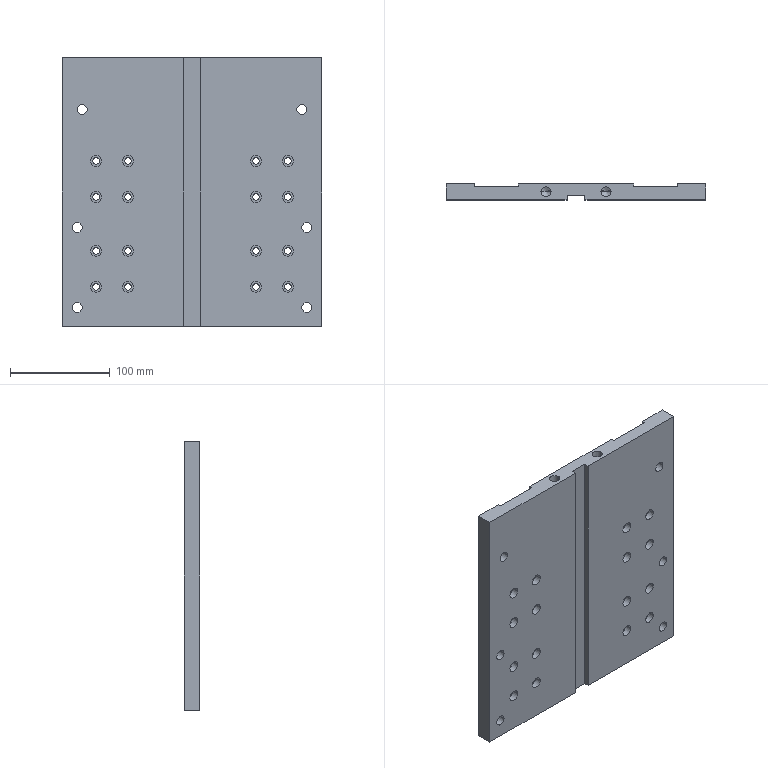Component | SolidWorks | NewTypeCurveBenderReinforcementSeatBasePlate-DoubleWheel-1 | 1 solid | 118 faces | box 260 x 16 x 269 mm | volume 1001671 mm3 | cylinder 80 | plane 34 | cone 4 | commonest cylinder face diameters 11 x32 6.6 x32 10.2 x16
build123d program:
from build123d import *

# Parameters (mm, degrees)
SKETCH1_W                                         = 119
SKETCH1_H                                         = 260
BOSS_EXTRUDE1_DEPTH                               = 16
M12_TAPPED_HOLE3_D                                = 10.2
SKETCH8_W                                         = 18
SKETCH8_H                                         = 4.5
SKETCH8_W_2                                       = 44
SKETCH8_H_2                                       = 6
CUT_EXTRUDE1_DEPTH                                = 177.966
BOSS_EXTRUDE2_DEPTH                               = 150
M12_TAPPED_HOLE1_D                                = 10.2
HOLE_SIZE_ACCORDING_TO_HEXAGON_SOCKET_D           = 6.6
HOLE_SIZE_ACCORDING_TO_HEXAGON_SOCKET_CBORE_D     = 11
HOLE_SIZE_ACCORDING_TO_HEXAGON_SOCKET_CBORE_DEPTH = 6.8
M12_TAPPED_HOLE2_D                                = 10.2
M12_TAPPED_HOLE2_DEPTH                            = 17.25
M12_TAPPED_HOLE2_TIP                              = 3.064


with BuildPart() as part:
    # Sketch1 → Boss-Extrude1 (new body)
    with BuildSketch(Plane(origin=(0, 0, 0), x_dir=(1, 0, 0), z_dir=(0, 1, 0))):
        Rectangle(SKETCH1_W, SKETCH1_H)
    extrude(amount=BOSS_EXTRUDE1_DEPTH)

    # M12 Tapped Hole3 (through all)
    with Locations(Plane(origin=(0, 16, 0), x_dir=(1, 0, 0), z_dir=(0, 1, 0))):
        with Locations((-40.5, 115), (39.5, 115), (39.5, -115), (-40.5, -115)):
            Hole(M12_TAPPED_HOLE3_D / 2)

    # Sketch8 → Cut-Extrude1 (cut, through all)
    with BuildSketch(Plane.ZY.offset(59.5)):
        with Locations((0, 13.75)):
            Rectangle(SKETCH8_W, SKETCH8_H)
        with Locations((-80, 0)):
            Rectangle(SKETCH8_W_2, SKETCH8_H_2)
        with Locations((80, 0)):
            Rectangle(SKETCH8_W_2, SKETCH8_H_2)
    extrude(amount=-CUT_EXTRUDE1_DEPTH, mode=Mode.SUBTRACT)

    # Sketch10 → Boss-Extrude2 (add)
    with BuildSketch(Plane(origin=(59.5, 0, 0), x_dir=(0, 0, -1), z_dir=(1, 0, 0))):
        Polygon((9, 11.5), (-9, 11.5), (-9, 16), (-130, 16), (-130, 0), (-102, 0), (-102, 3), (-58, 3), (-58, 0), (58, 0), (58, 3), (102, 3), (102, 0), (130, 0), (130, 16), (9, 16), align=None)
    extrude(amount=BOSS_EXTRUDE2_DEPTH)

    # M12 Tapped Hole1 (through all)
    with Locations(Plane(origin=(0, 16, 0), x_dir=(1, 0, 0), z_dir=(0, 1, 0))):
        with Locations((157.5, 110), (157.5, -110)):
            Hole(M12_TAPPED_HOLE1_D / 2)

    # Hole Size _ according to_ Hexagon Socket (through all)
    with Locations(Plane(origin=(0, 16, 0), x_dir=(1, 0, 0), z_dir=(0, 1, 0))):
        with Locations((-19.87, 96), (16.13, 96), (16.13, 64), (-19.87, 64), (-19.87, -64), (-19.87, -96), (16.13, -96), (16.13, -64), (70.13, 96), (106.13, 96), (106.13, 64), (70.13, 64), (70.13, -64), (106.13, -96), (70.13, -96), (106.13, -64)):
            CounterBoreHole(HOLE_SIZE_ACCORDING_TO_HEXAGON_SOCKET_D / 2, HOLE_SIZE_ACCORDING_TO_HEXAGON_SOCKET_CBORE_D / 2, HOLE_SIZE_ACCORDING_TO_HEXAGON_SOCKET_CBORE_DEPTH)

    # M12 Tapped Hole2
    with Locations(Plane(origin=(209.5, 0, 0), x_dir=(0, 0, -1), z_dir=(1, 0, 0))):
        with Locations((-30, 8), (30, 8)):
            Hole(M12_TAPPED_HOLE2_D / 2, depth=M12_TAPPED_HOLE2_DEPTH)
            with Locations((0, 0, -(M12_TAPPED_HOLE2_DEPTH + M12_TAPPED_HOLE2_TIP / 2))):  # 118° drill point
                Cone(0, M12_TAPPED_HOLE2_D / 2, M12_TAPPED_HOLE2_TIP, mode=Mode.SUBTRACT)


solid = part.part

# Placed as in the assembly
solid = solid.moved(Location((0, 36, 0.5), (180, 90, 0)))